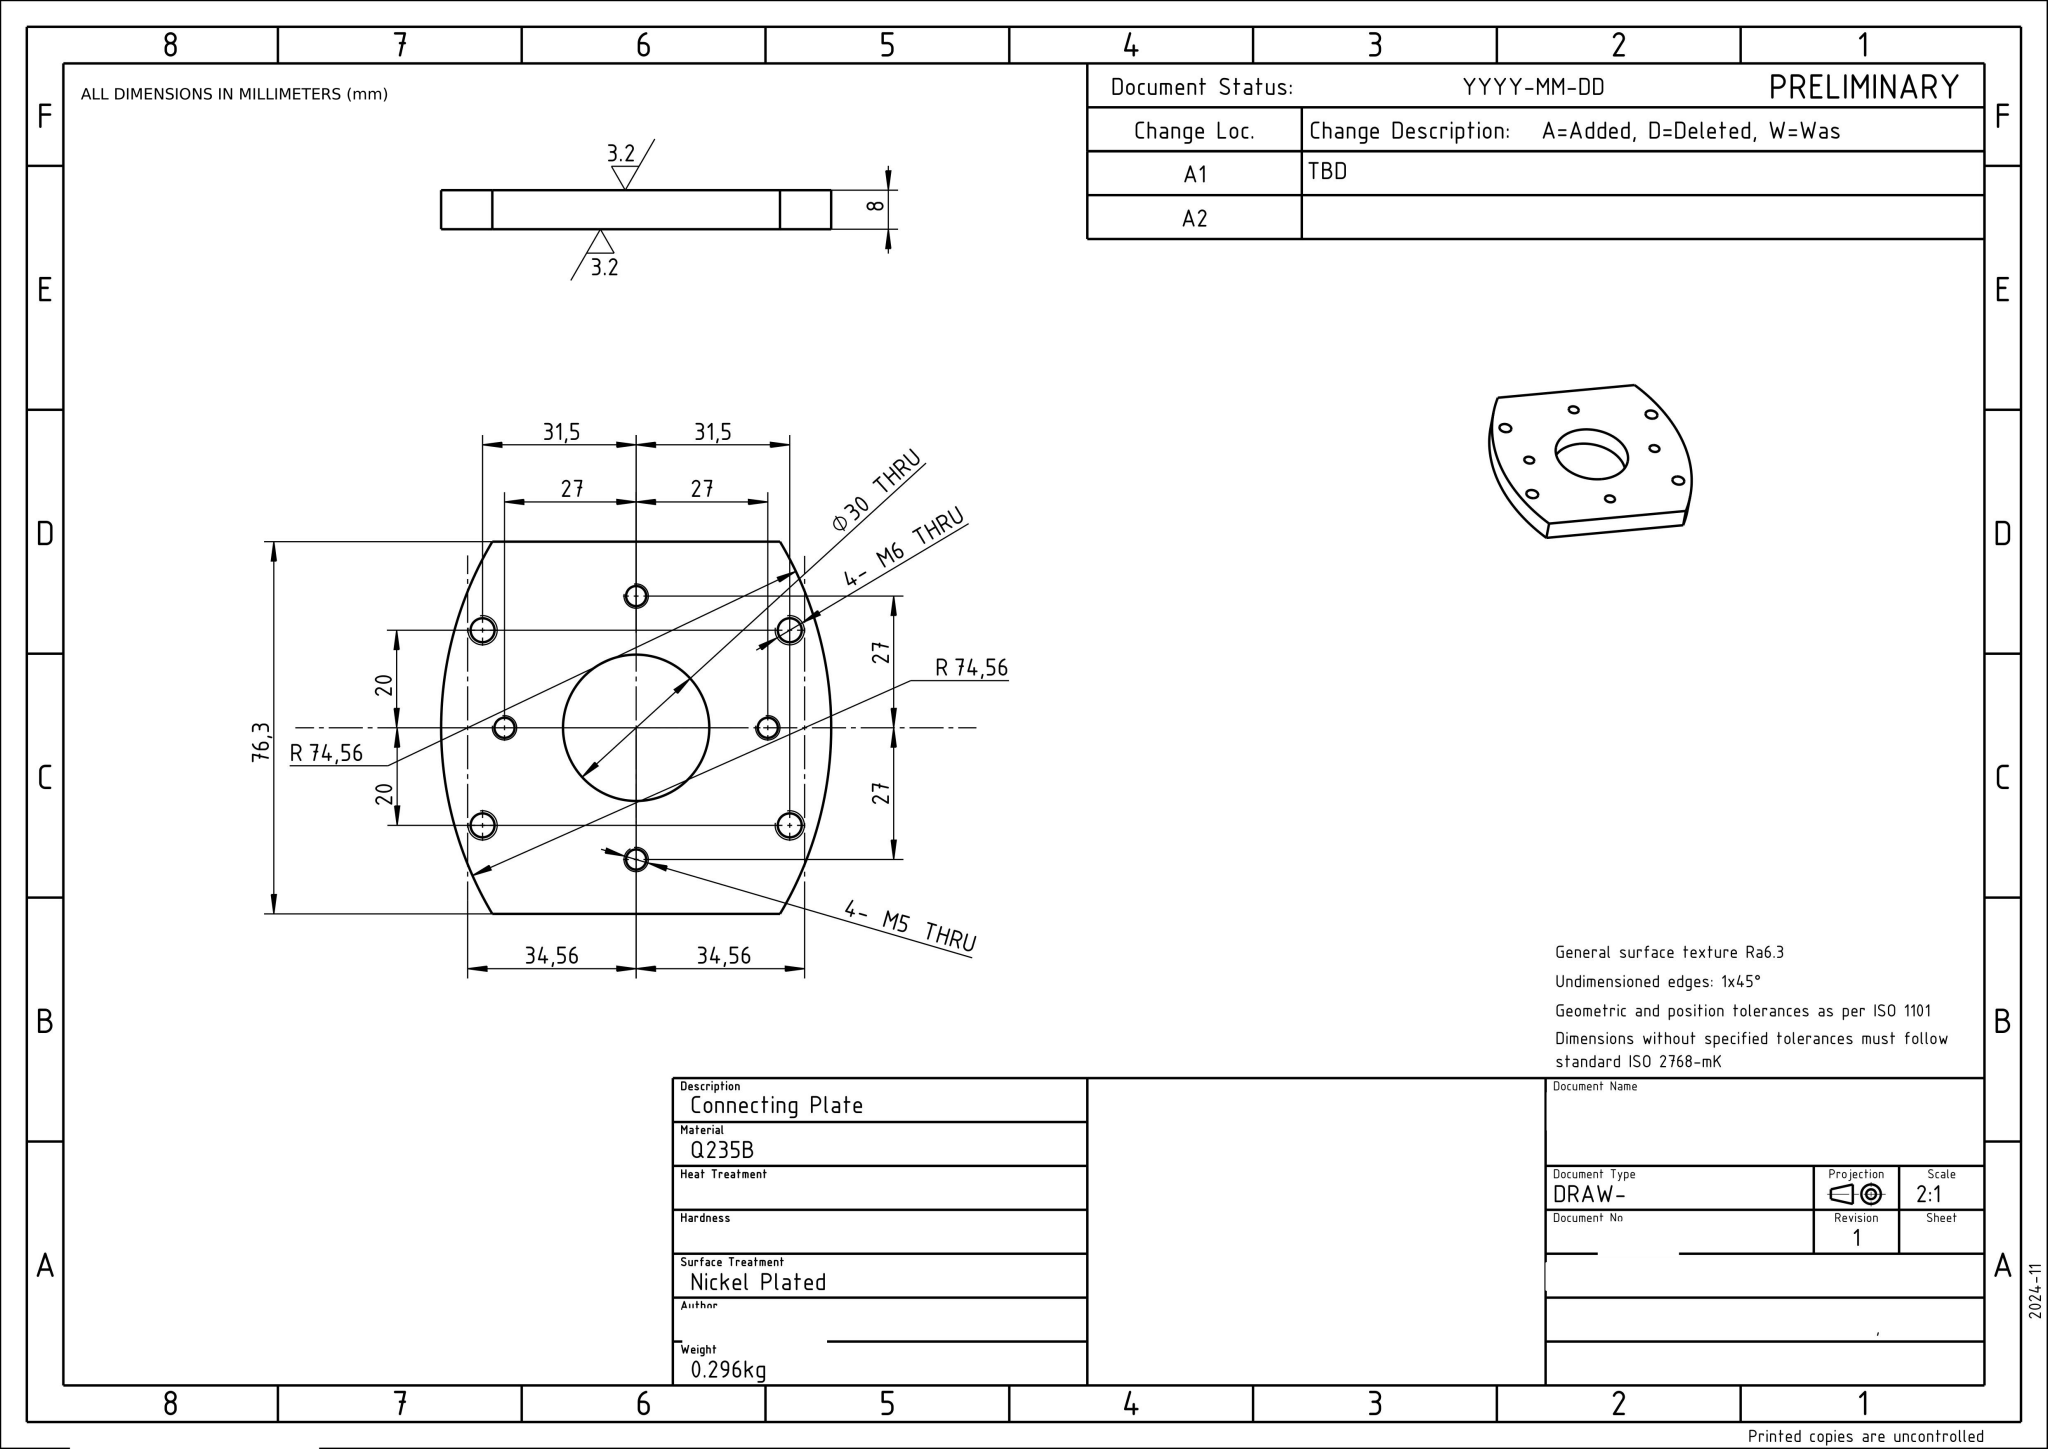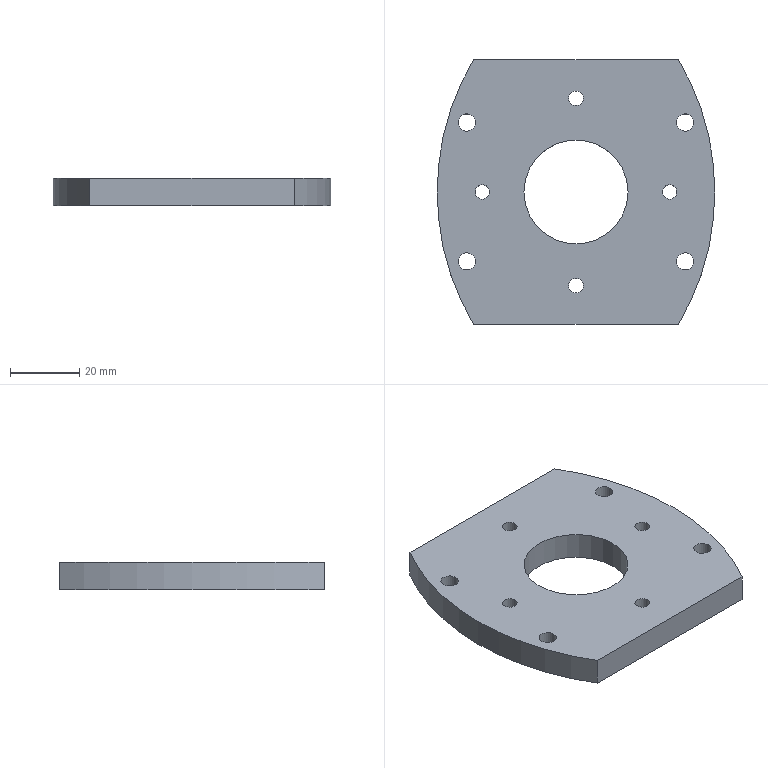Part | NX | mm | 1 solid | 15 faces | box 80 x 76.3 x 8 mm | volume 37961 mm3 | cylinder 11 | plane 4 | commonest cylinder face diameters 4.2 x4 5 x4 149.12 x2 30 x1
STEP:
#1=CARTESIAN_POINT('',(0.,0.,0.));
#2=DIRECTION('',(0.,0.,1.));
#3=DIRECTION('',(1.,0.,0.));
#4=AXIS2_PLACEMENT_3D('',#1,#2,#3);
#5=(LENGTH_UNIT()NAMED_UNIT(*)SI_UNIT(.MILLI.,.METRE.));
#6=UNCERTAINTY_MEASURE_WITH_UNIT(LENGTH_MEASURE(0.00002),#5,'','');
#7=(NAMED_UNIT(*)PLANE_ANGLE_UNIT()SI_UNIT($,.RADIAN.));
#8=PLANE_ANGLE_MEASURE_WITH_UNIT(PLANE_ANGLE_MEASURE(0.01745),#7);
#9=DIMENSIONAL_EXPONENTS(0.,0.,0.,0.,0.,0.,0.);
#10=(CONVERSION_BASED_UNIT('',#8)NAMED_UNIT(#9)PLANE_ANGLE_UNIT());
#11=(NAMED_UNIT(*)SI_UNIT($,.STERADIAN.)SOLID_ANGLE_UNIT());
#12=(GEOMETRIC_REPRESENTATION_CONTEXT(3)GLOBAL_UNCERTAINTY_ASSIGNED_CONTEXT((#6))GLOBAL_UNIT_ASSIGNED_CONTEXT((#5,#10,#11))REPRESENTATION_CONTEXT('',''));
#13=SHAPE_REPRESENTATION('',(#4),#12);
#14=CARTESIAN_POINT('',(-29.501,38.15,0.));
#15=VERTEX_POINT('',#14);
#16=CARTESIAN_POINT('',(-29.501,-38.15,0.));
#17=VERTEX_POINT('',#16);
#18=CARTESIAN_POINT('',(34.56,0.,0.));
#19=DIRECTION('',(0.,0.,1.));
#20=DIRECTION('',(1.,0.,0.));
#21=AXIS2_PLACEMENT_3D('',#18,#19,#20);
#22=CIRCLE('',#21,74.56);
#23=EDGE_CURVE('',#15,#17,#22,.T.);
#24=ORIENTED_EDGE('',*,*,#23,.T.);
#25=CARTESIAN_POINT('',(-29.501,-38.15,8.));
#26=VERTEX_POINT('',#25);
#27=CARTESIAN_POINT('',(-29.501,-38.15,8.));
#28=DIRECTION('',(0.,0.,-1.));
#29=VECTOR('',#28,1.);
#30=LINE('',#27,#29);
#31=EDGE_CURVE('',#26,#17,#30,.T.);
#32=ORIENTED_EDGE('',*,*,#31,.F.);
#33=CARTESIAN_POINT('',(-29.501,38.15,8.));
#34=VERTEX_POINT('',#33);
#35=CARTESIAN_POINT('',(34.56,0.,8.));
#36=DIRECTION('',(0.,0.,1.));
#37=DIRECTION('',(1.,0.,0.));
#38=AXIS2_PLACEMENT_3D('',#35,#36,#37);
#39=CIRCLE('',#38,74.56);
#40=EDGE_CURVE('',#34,#26,#39,.T.);
#41=ORIENTED_EDGE('',*,*,#40,.F.);
#42=CARTESIAN_POINT('',(-29.501,38.15,8.));
#43=DIRECTION('',(0.,0.,-1.));
#44=VECTOR('',#43,1.);
#45=LINE('',#42,#44);
#46=EDGE_CURVE('',#34,#15,#45,.T.);
#47=ORIENTED_EDGE('',*,*,#46,.T.);
#48=EDGE_LOOP('',(#24,#32,#41,#47));
#49=FACE_OUTER_BOUND('',#48,.T.);
#50=CARTESIAN_POINT('',(34.56,0.,8.));
#51=DIRECTION('',(0.,0.,-1.));
#52=DIRECTION('',(-1.,0.,0.));
#53=AXIS2_PLACEMENT_3D('',#50,#51,#52);
#54=CYLINDRICAL_SURFACE('',#53,74.56);
#55=ADVANCED_FACE('',(#49),#54,.T.);
#56=CARTESIAN_POINT('',(29.501,-38.15,0.));
#57=VERTEX_POINT('',#56);
#58=CARTESIAN_POINT('',(-29.501,-38.15,0.));
#59=DIRECTION('',(1.,-0.,0.));
#60=VECTOR('',#59,1.);
#61=LINE('',#58,#60);
#62=EDGE_CURVE('',#17,#57,#61,.T.);
#63=ORIENTED_EDGE('',*,*,#62,.T.);
#64=CARTESIAN_POINT('',(29.501,-38.15,8.));
#65=VERTEX_POINT('',#64);
#66=CARTESIAN_POINT('',(29.501,-38.15,8.));
#67=DIRECTION('',(0.,0.,-1.));
#68=VECTOR('',#67,1.);
#69=LINE('',#66,#68);
#70=EDGE_CURVE('',#65,#57,#69,.T.);
#71=ORIENTED_EDGE('',*,*,#70,.F.);
#72=CARTESIAN_POINT('',(-29.501,-38.15,8.));
#73=DIRECTION('',(1.,-0.,0.));
#74=VECTOR('',#73,1.);
#75=LINE('',#72,#74);
#76=EDGE_CURVE('',#26,#65,#75,.T.);
#77=ORIENTED_EDGE('',*,*,#76,.F.);
#78=ORIENTED_EDGE('',*,*,#31,.T.);
#79=EDGE_LOOP('',(#63,#71,#77,#78));
#80=FACE_OUTER_BOUND('',#79,.T.);
#81=CARTESIAN_POINT('',(-29.501,-38.15,8.));
#82=DIRECTION('',(0.,1.,0.));
#83=DIRECTION('',(-1.,0.,0.));
#84=AXIS2_PLACEMENT_3D('',#81,#82,#83);
#85=PLANE('',#84);
#86=ADVANCED_FACE('',(#80),#85,.F.);
#87=CARTESIAN_POINT('',(29.501,38.15,0.));
#88=VERTEX_POINT('',#87);
#89=CARTESIAN_POINT('',(-34.56,0.,0.));
#90=DIRECTION('',(0.,0.,1.));
#91=DIRECTION('',(-1.,0.,0.));
#92=AXIS2_PLACEMENT_3D('',#89,#90,#91);
#93=CIRCLE('',#92,74.56);
#94=EDGE_CURVE('',#57,#88,#93,.T.);
#95=ORIENTED_EDGE('',*,*,#94,.T.);
#96=CARTESIAN_POINT('',(29.501,38.15,8.));
#97=VERTEX_POINT('',#96);
#98=CARTESIAN_POINT('',(29.501,38.15,8.));
#99=DIRECTION('',(0.,0.,-1.));
#100=VECTOR('',#99,1.);
#101=LINE('',#98,#100);
#102=EDGE_CURVE('',#97,#88,#101,.T.);
#103=ORIENTED_EDGE('',*,*,#102,.F.);
#104=CARTESIAN_POINT('',(-34.56,0.,8.));
#105=DIRECTION('',(0.,0.,1.));
#106=DIRECTION('',(-1.,0.,0.));
#107=AXIS2_PLACEMENT_3D('',#104,#105,#106);
#108=CIRCLE('',#107,74.56);
#109=EDGE_CURVE('',#65,#97,#108,.T.);
#110=ORIENTED_EDGE('',*,*,#109,.F.);
#111=ORIENTED_EDGE('',*,*,#70,.T.);
#112=EDGE_LOOP('',(#95,#103,#110,#111));
#113=FACE_OUTER_BOUND('',#112,.T.);
#114=CARTESIAN_POINT('',(-34.56,0.,8.));
#115=DIRECTION('',(0.,0.,-1.));
#116=DIRECTION('',(-1.,0.,0.));
#117=AXIS2_PLACEMENT_3D('',#114,#115,#116);
#118=CYLINDRICAL_SURFACE('',#117,74.56);
#119=ADVANCED_FACE('',(#113),#118,.T.);
#120=CARTESIAN_POINT('',(29.501,38.15,0.));
#121=DIRECTION('',(-1.,0.,0.));
#122=VECTOR('',#121,1.);
#123=LINE('',#120,#122);
#124=EDGE_CURVE('',#88,#15,#123,.T.);
#125=ORIENTED_EDGE('',*,*,#124,.T.);
#126=ORIENTED_EDGE('',*,*,#46,.F.);
#127=CARTESIAN_POINT('',(29.501,38.15,8.));
#128=DIRECTION('',(-1.,0.,0.));
#129=VECTOR('',#128,1.);
#130=LINE('',#127,#129);
#131=EDGE_CURVE('',#97,#34,#130,.T.);
#132=ORIENTED_EDGE('',*,*,#131,.F.);
#133=ORIENTED_EDGE('',*,*,#102,.T.);
#134=EDGE_LOOP('',(#125,#126,#132,#133));
#135=FACE_OUTER_BOUND('',#134,.T.);
#136=CARTESIAN_POINT('',(29.501,38.15,8.));
#137=DIRECTION('',(0.,-1.,0.));
#138=DIRECTION('',(0.,0.,-1.));
#139=AXIS2_PLACEMENT_3D('',#136,#137,#138);
#140=PLANE('',#139);
#141=ADVANCED_FACE('',(#135),#140,.F.);
#142=CARTESIAN_POINT('',(15.,0.,8.));
#143=VERTEX_POINT('',#142);
#144=CARTESIAN_POINT('',(0.,0.,8.));
#145=DIRECTION('',(0.,0.,1.));
#146=DIRECTION('',(1.,0.,0.));
#147=AXIS2_PLACEMENT_3D('',#144,#145,#146);
#148=CIRCLE('',#147,15.);
#149=EDGE_CURVE('',#143,#143,#148,.T.);
#150=ORIENTED_EDGE('',*,*,#149,.T.);
#151=EDGE_LOOP('',(#150));
#152=FACE_BOUND('',#151,.T.);
#153=CARTESIAN_POINT('',(15.,0.,0.));
#154=VERTEX_POINT('',#153);
#155=CARTESIAN_POINT('',(0.,0.,0.));
#156=DIRECTION('',(0.,0.,1.));
#157=DIRECTION('',(1.,0.,0.));
#158=AXIS2_PLACEMENT_3D('',#155,#156,#157);
#159=CIRCLE('',#158,15.);
#160=EDGE_CURVE('',#154,#154,#159,.T.);
#161=ORIENTED_EDGE('',*,*,#160,.F.);
#162=EDGE_LOOP('',(#161));
#163=FACE_BOUND('',#162,.T.);
#164=CARTESIAN_POINT('',(0.,0.,8.));
#165=DIRECTION('',(0.,0.,-1.));
#166=DIRECTION('',(-1.,0.,0.));
#167=AXIS2_PLACEMENT_3D('',#164,#165,#166);
#168=CYLINDRICAL_SURFACE('',#167,15.);
#169=ADVANCED_FACE('',(#152,#163),#168,.F.);
#170=CARTESIAN_POINT('',(34.,20.,8.));
#171=VERTEX_POINT('',#170);
#172=CARTESIAN_POINT('',(31.5,20.,8.));
#173=DIRECTION('',(0.,0.,1.));
#174=DIRECTION('',(1.,0.,0.));
#175=AXIS2_PLACEMENT_3D('',#172,#173,#174);
#176=CIRCLE('',#175,2.5);
#177=EDGE_CURVE('',#171,#171,#176,.T.);
#178=ORIENTED_EDGE('',*,*,#177,.F.);
#179=EDGE_LOOP('',(#178));
#180=FACE_BOUND('',#179,.T.);
#181=CARTESIAN_POINT('',(34.,-20.,8.));
#182=VERTEX_POINT('',#181);
#183=CARTESIAN_POINT('',(31.5,-20.,8.));
#184=DIRECTION('',(0.,0.,1.));
#185=DIRECTION('',(1.,0.,0.));
#186=AXIS2_PLACEMENT_3D('',#183,#184,#185);
#187=CIRCLE('',#186,2.5);
#188=EDGE_CURVE('',#182,#182,#187,.T.);
#189=ORIENTED_EDGE('',*,*,#188,.F.);
#190=EDGE_LOOP('',(#189));
#191=FACE_BOUND('',#190,.T.);
#192=CARTESIAN_POINT('',(-29.,20.,8.));
#193=VERTEX_POINT('',#192);
#194=CARTESIAN_POINT('',(-31.5,20.,8.));
#195=DIRECTION('',(0.,0.,1.));
#196=DIRECTION('',(1.,0.,0.));
#197=AXIS2_PLACEMENT_3D('',#194,#195,#196);
#198=CIRCLE('',#197,2.5);
#199=EDGE_CURVE('',#193,#193,#198,.T.);
#200=ORIENTED_EDGE('',*,*,#199,.F.);
#201=EDGE_LOOP('',(#200));
#202=FACE_BOUND('',#201,.T.);
#203=CARTESIAN_POINT('',(-29.,-20.,8.));
#204=VERTEX_POINT('',#203);
#205=CARTESIAN_POINT('',(-31.5,-20.,8.));
#206=DIRECTION('',(0.,0.,1.));
#207=DIRECTION('',(1.,0.,0.));
#208=AXIS2_PLACEMENT_3D('',#205,#206,#207);
#209=CIRCLE('',#208,2.5);
#210=EDGE_CURVE('',#204,#204,#209,.T.);
#211=ORIENTED_EDGE('',*,*,#210,.F.);
#212=EDGE_LOOP('',(#211));
#213=FACE_BOUND('',#212,.T.);
#214=CARTESIAN_POINT('',(29.1,0.,8.));
#215=VERTEX_POINT('',#214);
#216=CARTESIAN_POINT('',(27.,0.,8.));
#217=DIRECTION('',(0.,0.,1.));
#218=DIRECTION('',(1.,0.,0.));
#219=AXIS2_PLACEMENT_3D('',#216,#217,#218);
#220=CIRCLE('',#219,2.1);
#221=EDGE_CURVE('',#215,#215,#220,.T.);
#222=ORIENTED_EDGE('',*,*,#221,.F.);
#223=EDGE_LOOP('',(#222));
#224=FACE_BOUND('',#223,.T.);
#225=CARTESIAN_POINT('',(2.1,27.,8.));
#226=VERTEX_POINT('',#225);
#227=CARTESIAN_POINT('',(0.,27.,8.));
#228=DIRECTION('',(0.,0.,1.));
#229=DIRECTION('',(1.,0.,0.));
#230=AXIS2_PLACEMENT_3D('',#227,#228,#229);
#231=CIRCLE('',#230,2.1);
#232=EDGE_CURVE('',#226,#226,#231,.T.);
#233=ORIENTED_EDGE('',*,*,#232,.F.);
#234=EDGE_LOOP('',(#233));
#235=FACE_BOUND('',#234,.T.);
#236=CARTESIAN_POINT('',(2.1,-27.,8.));
#237=VERTEX_POINT('',#236);
#238=CARTESIAN_POINT('',(-0.,-27.,8.));
#239=DIRECTION('',(0.,0.,1.));
#240=DIRECTION('',(1.,0.,0.));
#241=AXIS2_PLACEMENT_3D('',#238,#239,#240);
#242=CIRCLE('',#241,2.1);
#243=EDGE_CURVE('',#237,#237,#242,.T.);
#244=ORIENTED_EDGE('',*,*,#243,.F.);
#245=EDGE_LOOP('',(#244));
#246=FACE_BOUND('',#245,.T.);
#247=CARTESIAN_POINT('',(-24.9,0.,8.));
#248=VERTEX_POINT('',#247);
#249=CARTESIAN_POINT('',(-27.,0.,8.));
#250=DIRECTION('',(0.,0.,1.));
#251=DIRECTION('',(1.,0.,0.));
#252=AXIS2_PLACEMENT_3D('',#249,#250,#251);
#253=CIRCLE('',#252,2.1);
#254=EDGE_CURVE('',#248,#248,#253,.T.);
#255=ORIENTED_EDGE('',*,*,#254,.F.);
#256=EDGE_LOOP('',(#255));
#257=FACE_BOUND('',#256,.T.);
#258=ORIENTED_EDGE('',*,*,#40,.T.);
#259=ORIENTED_EDGE('',*,*,#76,.T.);
#260=ORIENTED_EDGE('',*,*,#109,.T.);
#261=ORIENTED_EDGE('',*,*,#131,.T.);
#262=EDGE_LOOP('',(#258,#259,#260,#261));
#263=FACE_BOUND('',#262,.T.);
#264=ORIENTED_EDGE('',*,*,#149,.F.);
#265=EDGE_LOOP('',(#264));
#266=FACE_BOUND('',#265,.T.);
#267=CARTESIAN_POINT('',(34.56,0.,8.));
#268=DIRECTION('',(0.,0.,1.));
#269=DIRECTION('',(1.,0.,0.));
#270=AXIS2_PLACEMENT_3D('',#267,#268,#269);
#271=PLANE('',#270);
#272=ADVANCED_FACE('',(#180,#191,#202,#213,#224,#235,#246,#257,#263,#266),#271,.T.);
#273=CARTESIAN_POINT('',(34.,20.,0.));
#274=VERTEX_POINT('',#273);
#275=CARTESIAN_POINT('',(31.5,20.,0.));
#276=DIRECTION('',(0.,0.,1.));
#277=DIRECTION('',(1.,0.,0.));
#278=AXIS2_PLACEMENT_3D('',#275,#276,#277);
#279=CIRCLE('',#278,2.5);
#280=EDGE_CURVE('',#274,#274,#279,.T.);
#281=ORIENTED_EDGE('',*,*,#280,.T.);
#282=EDGE_LOOP('',(#281));
#283=FACE_BOUND('',#282,.T.);
#284=CARTESIAN_POINT('',(34.,-20.,0.));
#285=VERTEX_POINT('',#284);
#286=CARTESIAN_POINT('',(31.5,-20.,0.));
#287=DIRECTION('',(0.,0.,1.));
#288=DIRECTION('',(1.,0.,0.));
#289=AXIS2_PLACEMENT_3D('',#286,#287,#288);
#290=CIRCLE('',#289,2.5);
#291=EDGE_CURVE('',#285,#285,#290,.T.);
#292=ORIENTED_EDGE('',*,*,#291,.T.);
#293=EDGE_LOOP('',(#292));
#294=FACE_BOUND('',#293,.T.);
#295=CARTESIAN_POINT('',(-29.,20.,0.));
#296=VERTEX_POINT('',#295);
#297=CARTESIAN_POINT('',(-31.5,20.,0.));
#298=DIRECTION('',(0.,0.,1.));
#299=DIRECTION('',(1.,0.,0.));
#300=AXIS2_PLACEMENT_3D('',#297,#298,#299);
#301=CIRCLE('',#300,2.5);
#302=EDGE_CURVE('',#296,#296,#301,.T.);
#303=ORIENTED_EDGE('',*,*,#302,.T.);
#304=EDGE_LOOP('',(#303));
#305=FACE_BOUND('',#304,.T.);
#306=CARTESIAN_POINT('',(-29.,-20.,0.));
#307=VERTEX_POINT('',#306);
#308=CARTESIAN_POINT('',(-31.5,-20.,0.));
#309=DIRECTION('',(0.,0.,1.));
#310=DIRECTION('',(1.,0.,0.));
#311=AXIS2_PLACEMENT_3D('',#308,#309,#310);
#312=CIRCLE('',#311,2.5);
#313=EDGE_CURVE('',#307,#307,#312,.T.);
#314=ORIENTED_EDGE('',*,*,#313,.T.);
#315=EDGE_LOOP('',(#314));
#316=FACE_BOUND('',#315,.T.);
#317=CARTESIAN_POINT('',(29.1,0.,0.));
#318=VERTEX_POINT('',#317);
#319=CARTESIAN_POINT('',(27.,0.,0.));
#320=DIRECTION('',(0.,0.,1.));
#321=DIRECTION('',(1.,0.,0.));
#322=AXIS2_PLACEMENT_3D('',#319,#320,#321);
#323=CIRCLE('',#322,2.1);
#324=EDGE_CURVE('',#318,#318,#323,.T.);
#325=ORIENTED_EDGE('',*,*,#324,.T.);
#326=EDGE_LOOP('',(#325));
#327=FACE_BOUND('',#326,.T.);
#328=CARTESIAN_POINT('',(2.1,27.,0.));
#329=VERTEX_POINT('',#328);
#330=CARTESIAN_POINT('',(0.,27.,0.));
#331=DIRECTION('',(0.,0.,1.));
#332=DIRECTION('',(1.,0.,0.));
#333=AXIS2_PLACEMENT_3D('',#330,#331,#332);
#334=CIRCLE('',#333,2.1);
#335=EDGE_CURVE('',#329,#329,#334,.T.);
#336=ORIENTED_EDGE('',*,*,#335,.T.);
#337=EDGE_LOOP('',(#336));
#338=FACE_BOUND('',#337,.T.);
#339=CARTESIAN_POINT('',(2.1,-27.,0.));
#340=VERTEX_POINT('',#339);
#341=CARTESIAN_POINT('',(-0.,-27.,0.));
#342=DIRECTION('',(0.,0.,1.));
#343=DIRECTION('',(1.,0.,0.));
#344=AXIS2_PLACEMENT_3D('',#341,#342,#343);
#345=CIRCLE('',#344,2.1);
#346=EDGE_CURVE('',#340,#340,#345,.T.);
#347=ORIENTED_EDGE('',*,*,#346,.T.);
#348=EDGE_LOOP('',(#347));
#349=FACE_BOUND('',#348,.T.);
#350=CARTESIAN_POINT('',(-24.9,0.,0.));
#351=VERTEX_POINT('',#350);
#352=CARTESIAN_POINT('',(-27.,0.,0.));
#353=DIRECTION('',(0.,0.,1.));
#354=DIRECTION('',(1.,0.,0.));
#355=AXIS2_PLACEMENT_3D('',#352,#353,#354);
#356=CIRCLE('',#355,2.1);
#357=EDGE_CURVE('',#351,#351,#356,.T.);
#358=ORIENTED_EDGE('',*,*,#357,.T.);
#359=EDGE_LOOP('',(#358));
#360=FACE_BOUND('',#359,.T.);
#361=ORIENTED_EDGE('',*,*,#23,.F.);
#362=ORIENTED_EDGE('',*,*,#124,.F.);
#363=ORIENTED_EDGE('',*,*,#94,.F.);
#364=ORIENTED_EDGE('',*,*,#62,.F.);
#365=EDGE_LOOP('',(#361,#362,#363,#364));
#366=FACE_BOUND('',#365,.T.);
#367=ORIENTED_EDGE('',*,*,#160,.T.);
#368=EDGE_LOOP('',(#367));
#369=FACE_BOUND('',#368,.T.);
#370=CARTESIAN_POINT('',(34.56,0.,0.));
#371=DIRECTION('',(0.,0.,1.));
#372=DIRECTION('',(1.,0.,0.));
#373=AXIS2_PLACEMENT_3D('',#370,#371,#372);
#374=PLANE('',#373);
#375=ADVANCED_FACE('',(#283,#294,#305,#316,#327,#338,#349,#360,#366,#369),#374,.F.);
#376=ORIENTED_EDGE('',*,*,#254,.T.);
#377=EDGE_LOOP('',(#376));
#378=FACE_BOUND('',#377,.T.);
#379=ORIENTED_EDGE('',*,*,#357,.F.);
#380=EDGE_LOOP('',(#379));
#381=FACE_BOUND('',#380,.T.);
#382=CARTESIAN_POINT('',(-27.,0.,0.));
#383=DIRECTION('',(0.,0.,1.));
#384=DIRECTION('',(1.,0.,0.));
#385=AXIS2_PLACEMENT_3D('',#382,#383,#384);
#386=CYLINDRICAL_SURFACE('',#385,2.1);
#387=ADVANCED_FACE('',(#378,#381),#386,.F.);
#388=ORIENTED_EDGE('',*,*,#243,.T.);
#389=EDGE_LOOP('',(#388));
#390=FACE_BOUND('',#389,.T.);
#391=ORIENTED_EDGE('',*,*,#346,.F.);
#392=EDGE_LOOP('',(#391));
#393=FACE_BOUND('',#392,.T.);
#394=CARTESIAN_POINT('',(-0.,-27.,0.));
#395=DIRECTION('',(0.,0.,1.));
#396=DIRECTION('',(1.,0.,0.));
#397=AXIS2_PLACEMENT_3D('',#394,#395,#396);
#398=CYLINDRICAL_SURFACE('',#397,2.1);
#399=ADVANCED_FACE('',(#390,#393),#398,.F.);
#400=ORIENTED_EDGE('',*,*,#232,.T.);
#401=EDGE_LOOP('',(#400));
#402=FACE_BOUND('',#401,.T.);
#403=ORIENTED_EDGE('',*,*,#335,.F.);
#404=EDGE_LOOP('',(#403));
#405=FACE_BOUND('',#404,.T.);
#406=CARTESIAN_POINT('',(0.,27.,0.));
#407=DIRECTION('',(0.,0.,1.));
#408=DIRECTION('',(1.,0.,0.));
#409=AXIS2_PLACEMENT_3D('',#406,#407,#408);
#410=CYLINDRICAL_SURFACE('',#409,2.1);
#411=ADVANCED_FACE('',(#402,#405),#410,.F.);
#412=ORIENTED_EDGE('',*,*,#221,.T.);
#413=EDGE_LOOP('',(#412));
#414=FACE_BOUND('',#413,.T.);
#415=ORIENTED_EDGE('',*,*,#324,.F.);
#416=EDGE_LOOP('',(#415));
#417=FACE_BOUND('',#416,.T.);
#418=CARTESIAN_POINT('',(27.,0.,0.));
#419=DIRECTION('',(0.,0.,1.));
#420=DIRECTION('',(1.,0.,0.));
#421=AXIS2_PLACEMENT_3D('',#418,#419,#420);
#422=CYLINDRICAL_SURFACE('',#421,2.1);
#423=ADVANCED_FACE('',(#414,#417),#422,.F.);
#424=ORIENTED_EDGE('',*,*,#210,.T.);
#425=EDGE_LOOP('',(#424));
#426=FACE_BOUND('',#425,.T.);
#427=ORIENTED_EDGE('',*,*,#313,.F.);
#428=EDGE_LOOP('',(#427));
#429=FACE_BOUND('',#428,.T.);
#430=CARTESIAN_POINT('',(-31.5,-20.,0.));
#431=DIRECTION('',(0.,0.,1.));
#432=DIRECTION('',(1.,0.,0.));
#433=AXIS2_PLACEMENT_3D('',#430,#431,#432);
#434=CYLINDRICAL_SURFACE('',#433,2.5);
#435=ADVANCED_FACE('',(#426,#429),#434,.F.);
#436=ORIENTED_EDGE('',*,*,#199,.T.);
#437=EDGE_LOOP('',(#436));
#438=FACE_BOUND('',#437,.T.);
#439=ORIENTED_EDGE('',*,*,#302,.F.);
#440=EDGE_LOOP('',(#439));
#441=FACE_BOUND('',#440,.T.);
#442=CARTESIAN_POINT('',(-31.5,20.,0.));
#443=DIRECTION('',(0.,0.,1.));
#444=DIRECTION('',(1.,0.,0.));
#445=AXIS2_PLACEMENT_3D('',#442,#443,#444);
#446=CYLINDRICAL_SURFACE('',#445,2.5);
#447=ADVANCED_FACE('',(#438,#441),#446,.F.);
#448=ORIENTED_EDGE('',*,*,#188,.T.);
#449=EDGE_LOOP('',(#448));
#450=FACE_BOUND('',#449,.T.);
#451=ORIENTED_EDGE('',*,*,#291,.F.);
#452=EDGE_LOOP('',(#451));
#453=FACE_BOUND('',#452,.T.);
#454=CARTESIAN_POINT('',(31.5,-20.,0.));
#455=DIRECTION('',(0.,0.,1.));
#456=DIRECTION('',(1.,0.,0.));
#457=AXIS2_PLACEMENT_3D('',#454,#455,#456);
#458=CYLINDRICAL_SURFACE('',#457,2.5);
#459=ADVANCED_FACE('',(#450,#453),#458,.F.);
#460=ORIENTED_EDGE('',*,*,#177,.T.);
#461=EDGE_LOOP('',(#460));
#462=FACE_BOUND('',#461,.T.);
#463=ORIENTED_EDGE('',*,*,#280,.F.);
#464=EDGE_LOOP('',(#463));
#465=FACE_BOUND('',#464,.T.);
#466=CARTESIAN_POINT('',(31.5,20.,0.));
#467=DIRECTION('',(0.,0.,1.));
#468=DIRECTION('',(1.,0.,0.));
#469=AXIS2_PLACEMENT_3D('',#466,#467,#468);
#470=CYLINDRICAL_SURFACE('',#469,2.5);
#471=ADVANCED_FACE('',(#462,#465),#470,.F.);
#472=CLOSED_SHELL('',(#55,#86,#119,#141,#169,#272,#375,#387,#399,#411,#423,#435,#447,#459,#471));
#473=MANIFOLD_SOLID_BREP('',#472);
#474=ADVANCED_BREP_SHAPE_REPRESENTATION('',(#473),#12);
#475=SHAPE_REPRESENTATION_RELATIONSHIP('','',#13,#474);
#476=PRESENTATION_LAYER_ASSIGNMENT('','',(#473));
#477=COLOUR_RGB('',0.4,0.8,1.);
#478=FILL_AREA_STYLE_COLOUR('',#477);
#479=FILL_AREA_STYLE('',(#478));
#480=SURFACE_STYLE_FILL_AREA(#479);
#481=SURFACE_SIDE_STYLE('',(#480));
#482=SURFACE_STYLE_USAGE(.BOTH.,#481);
#483=PRESENTATION_STYLE_ASSIGNMENT((#482));
#484=STYLED_ITEM('',(#483),#473);
#485=MECHANICAL_DESIGN_GEOMETRIC_PRESENTATION_REPRESENTATION('',(#484),#12);